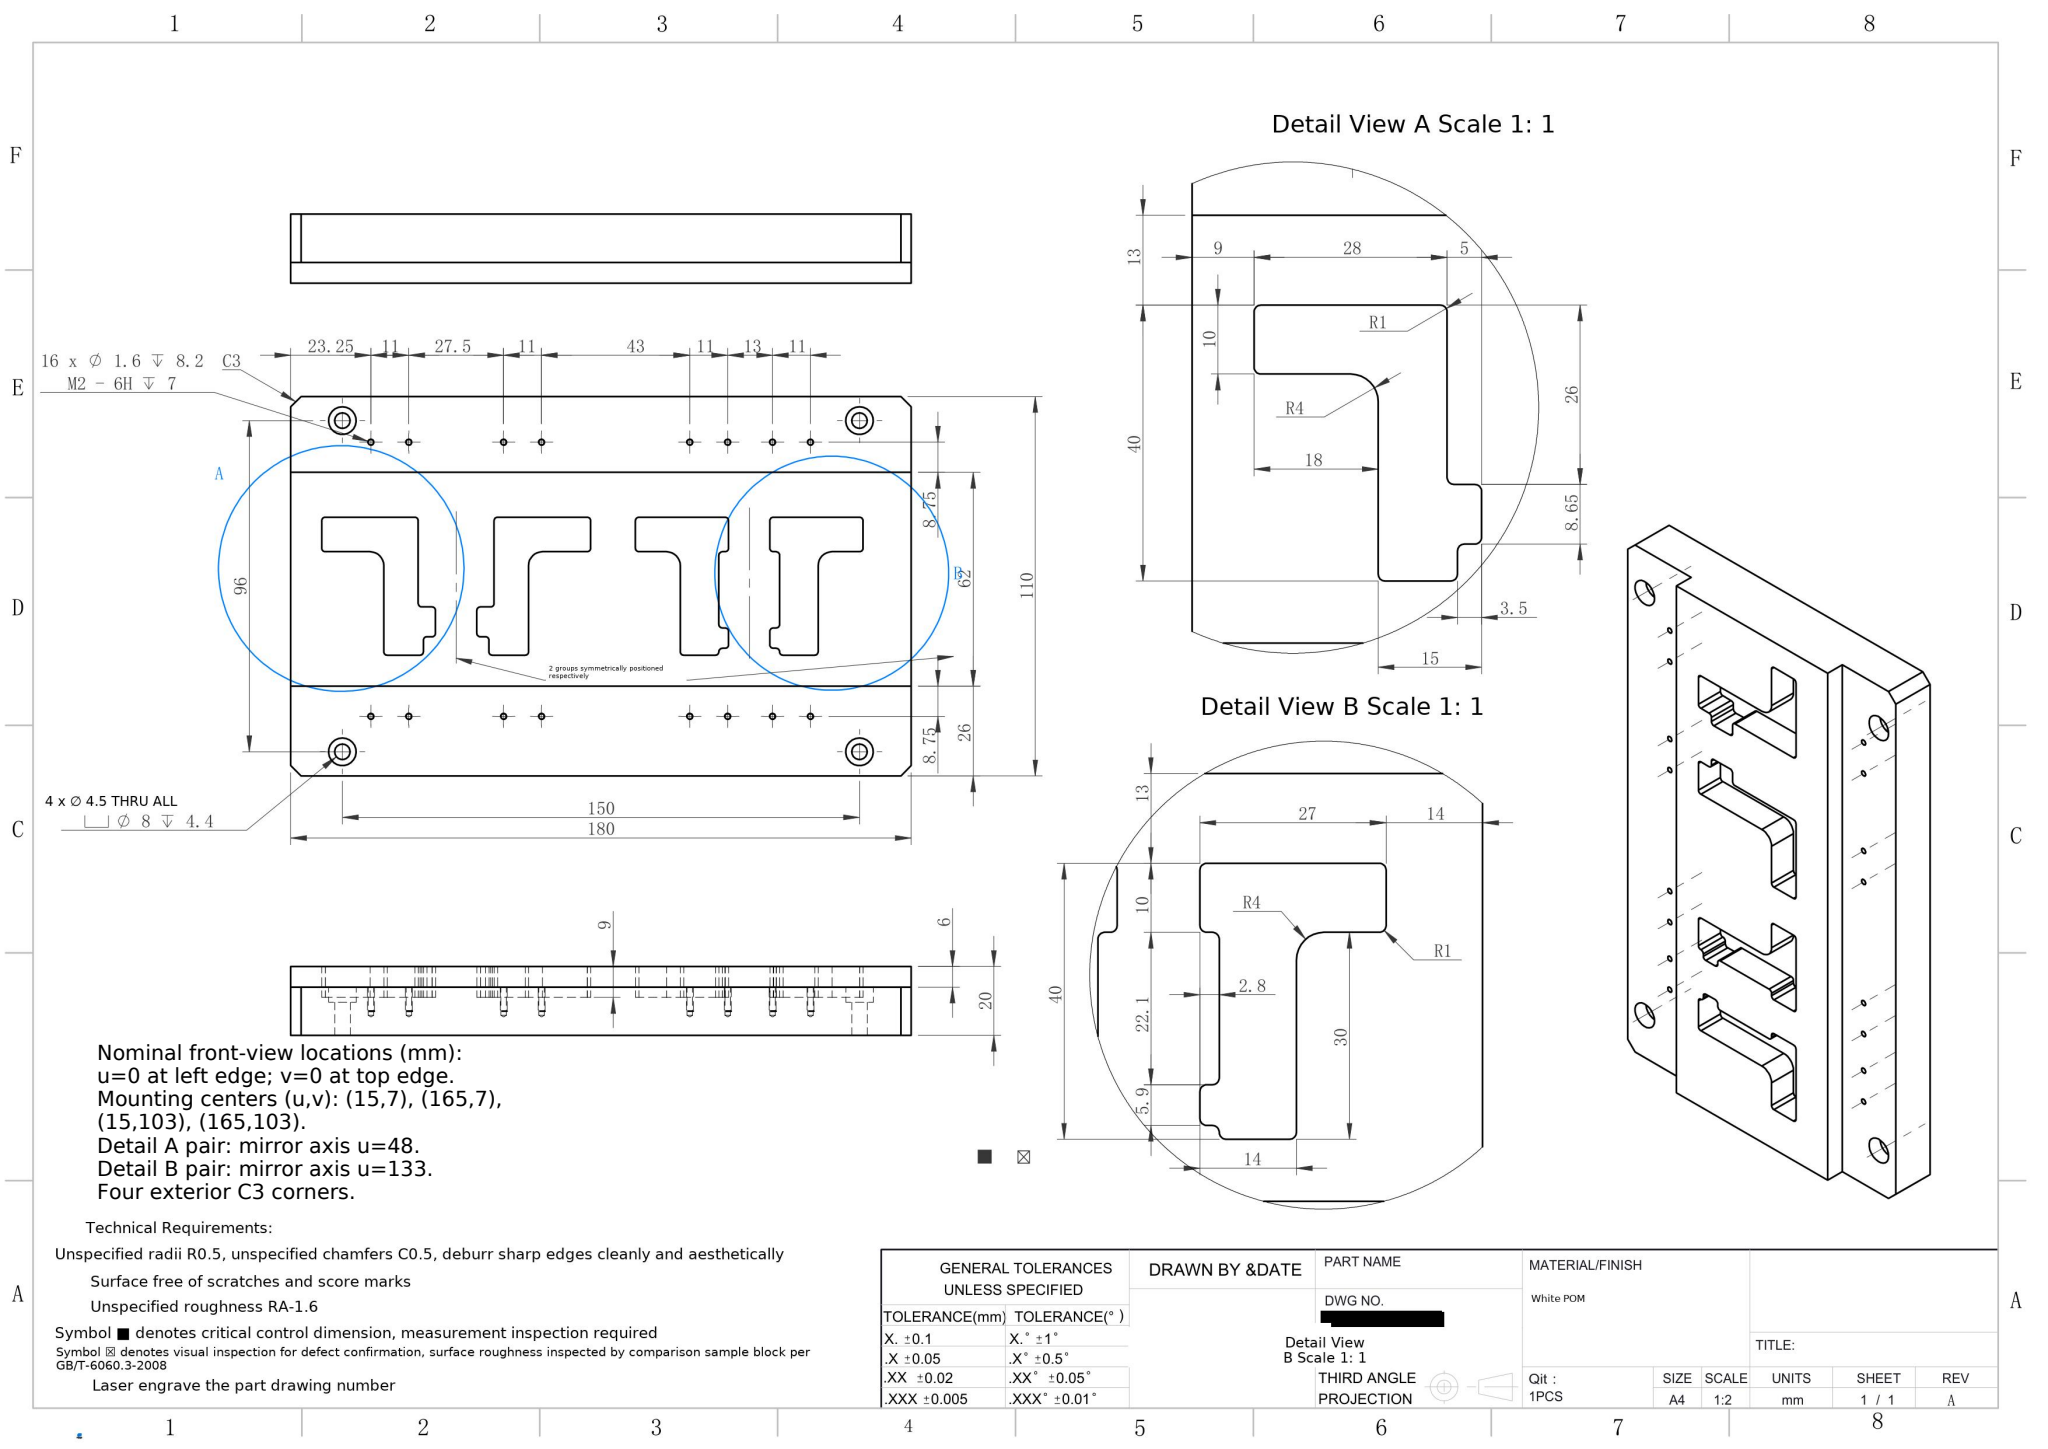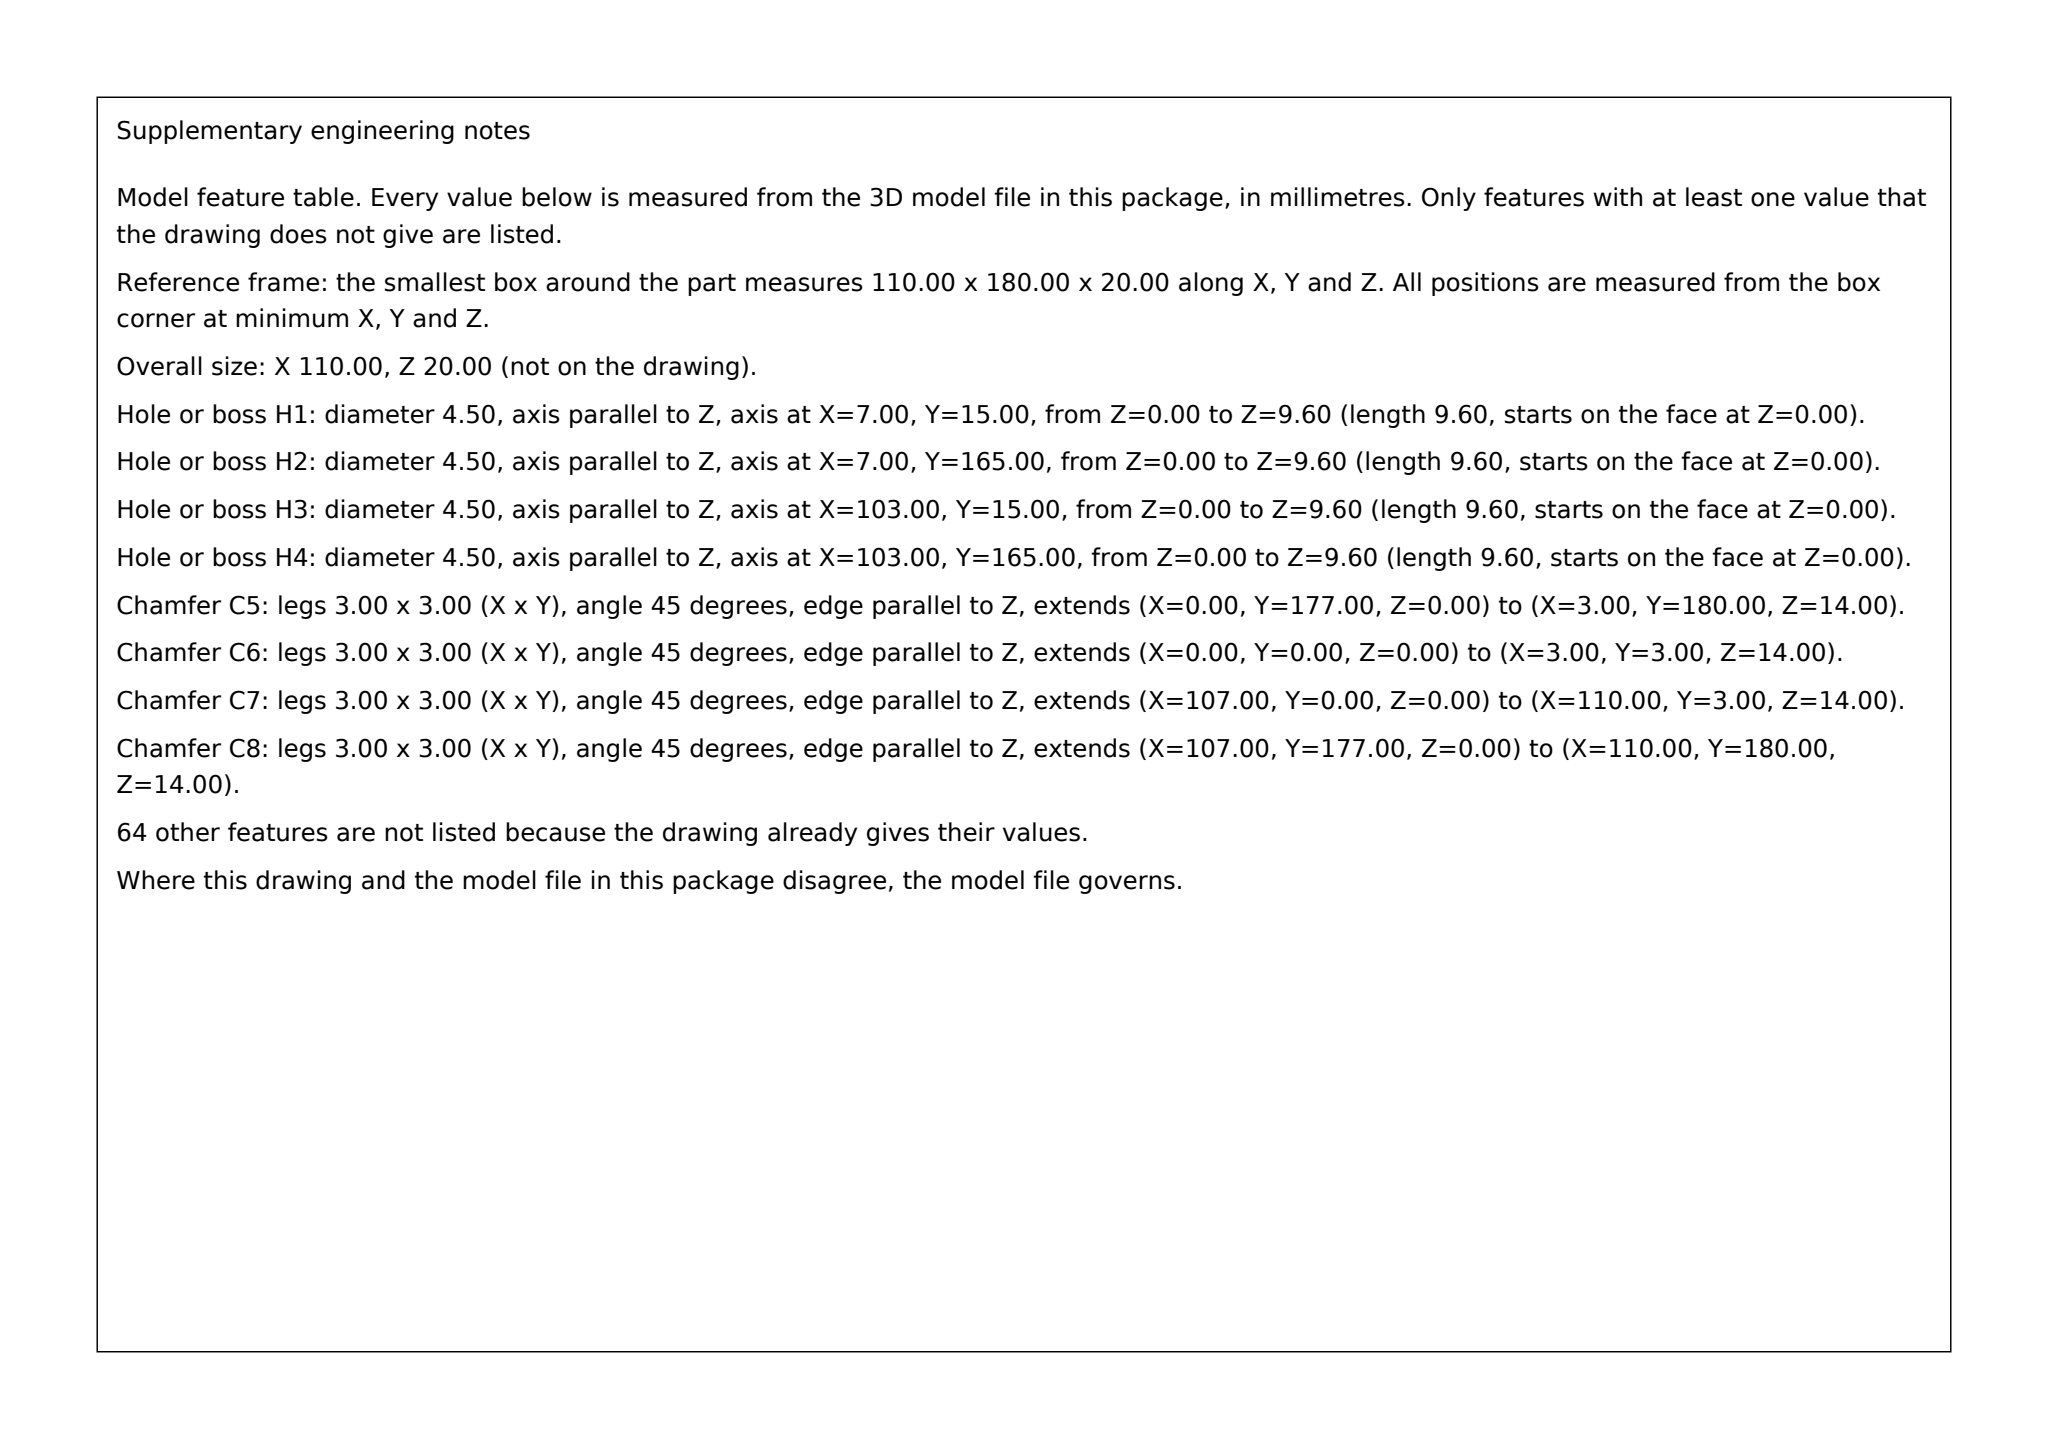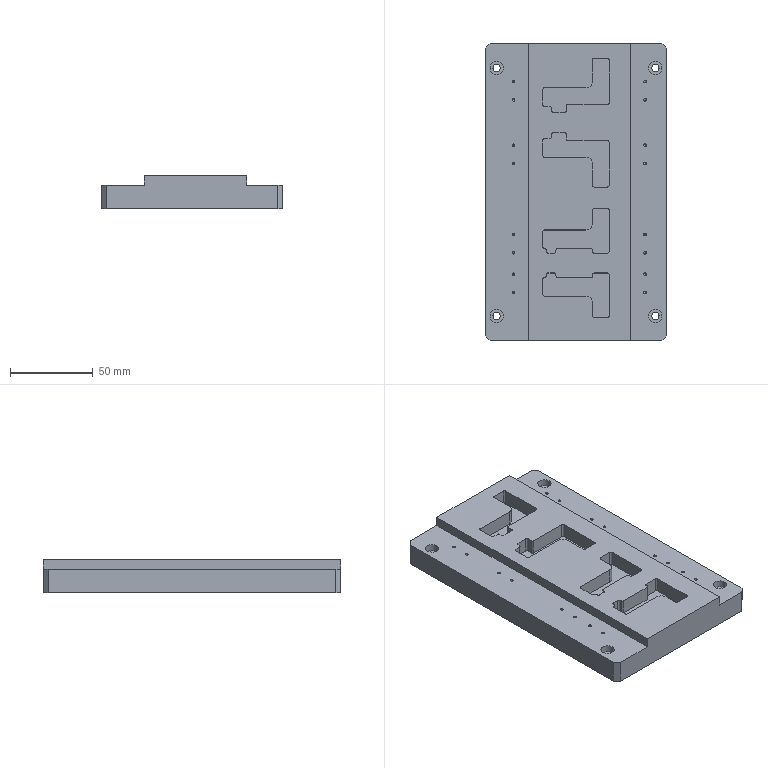Part | SolidWorks | mm | material White POM | 1 solid | 188 faces | box 110 x 180 x 20 mm | volume 319490 mm3 | cylinder 92 | plane 64 | cone 32 | commonest cylinder face diameters 2 x40 1.6 x32 8 x12 4.5 x8